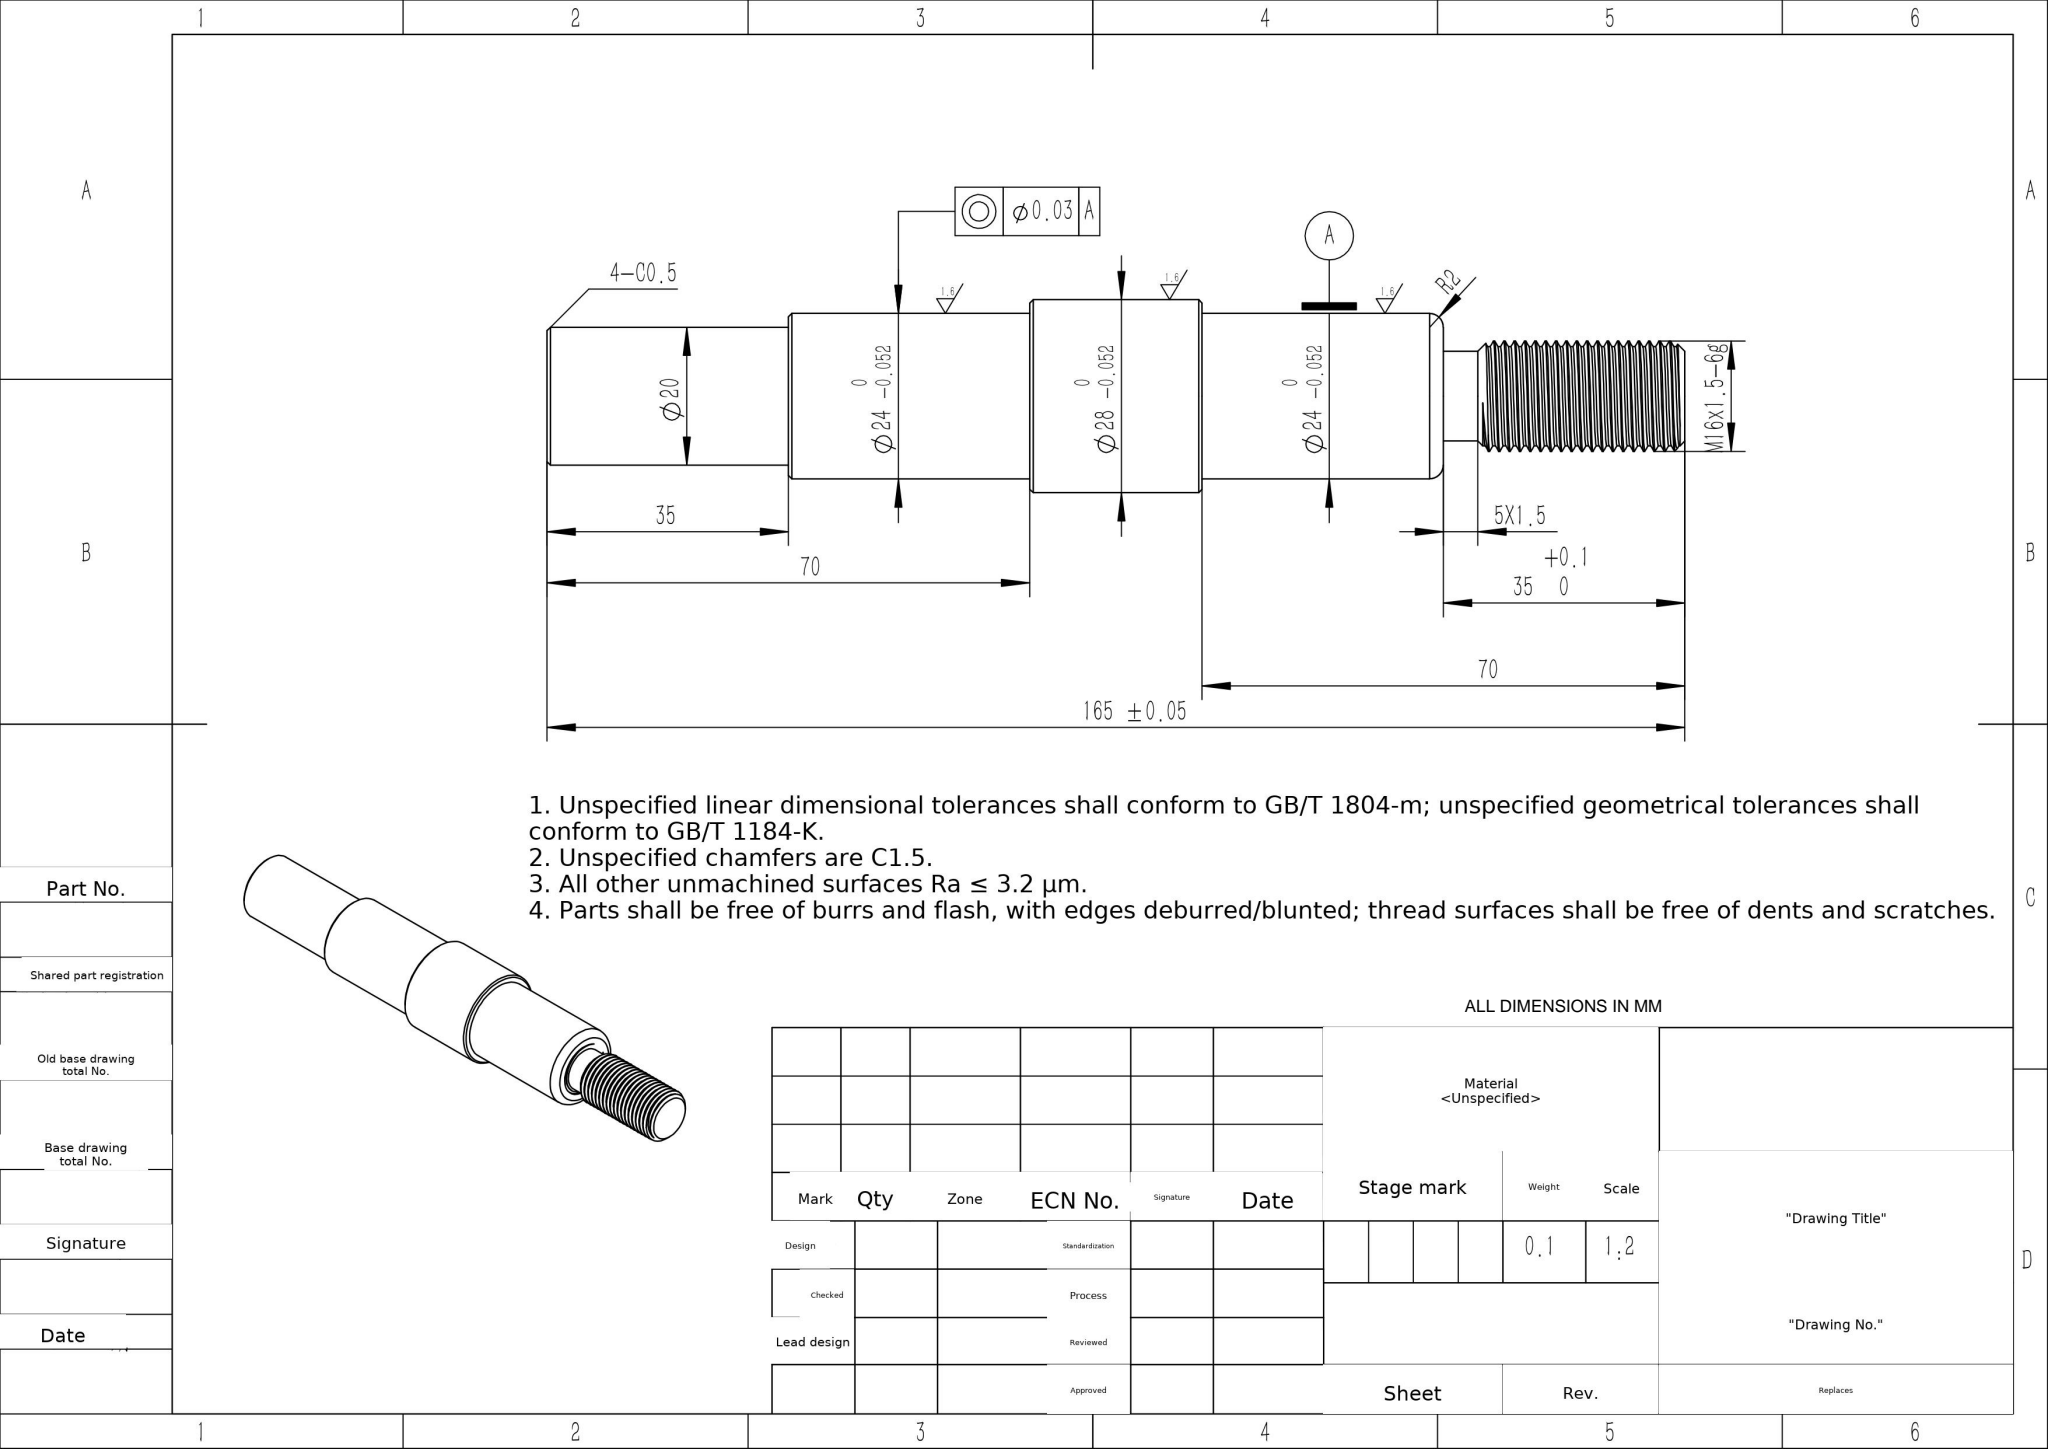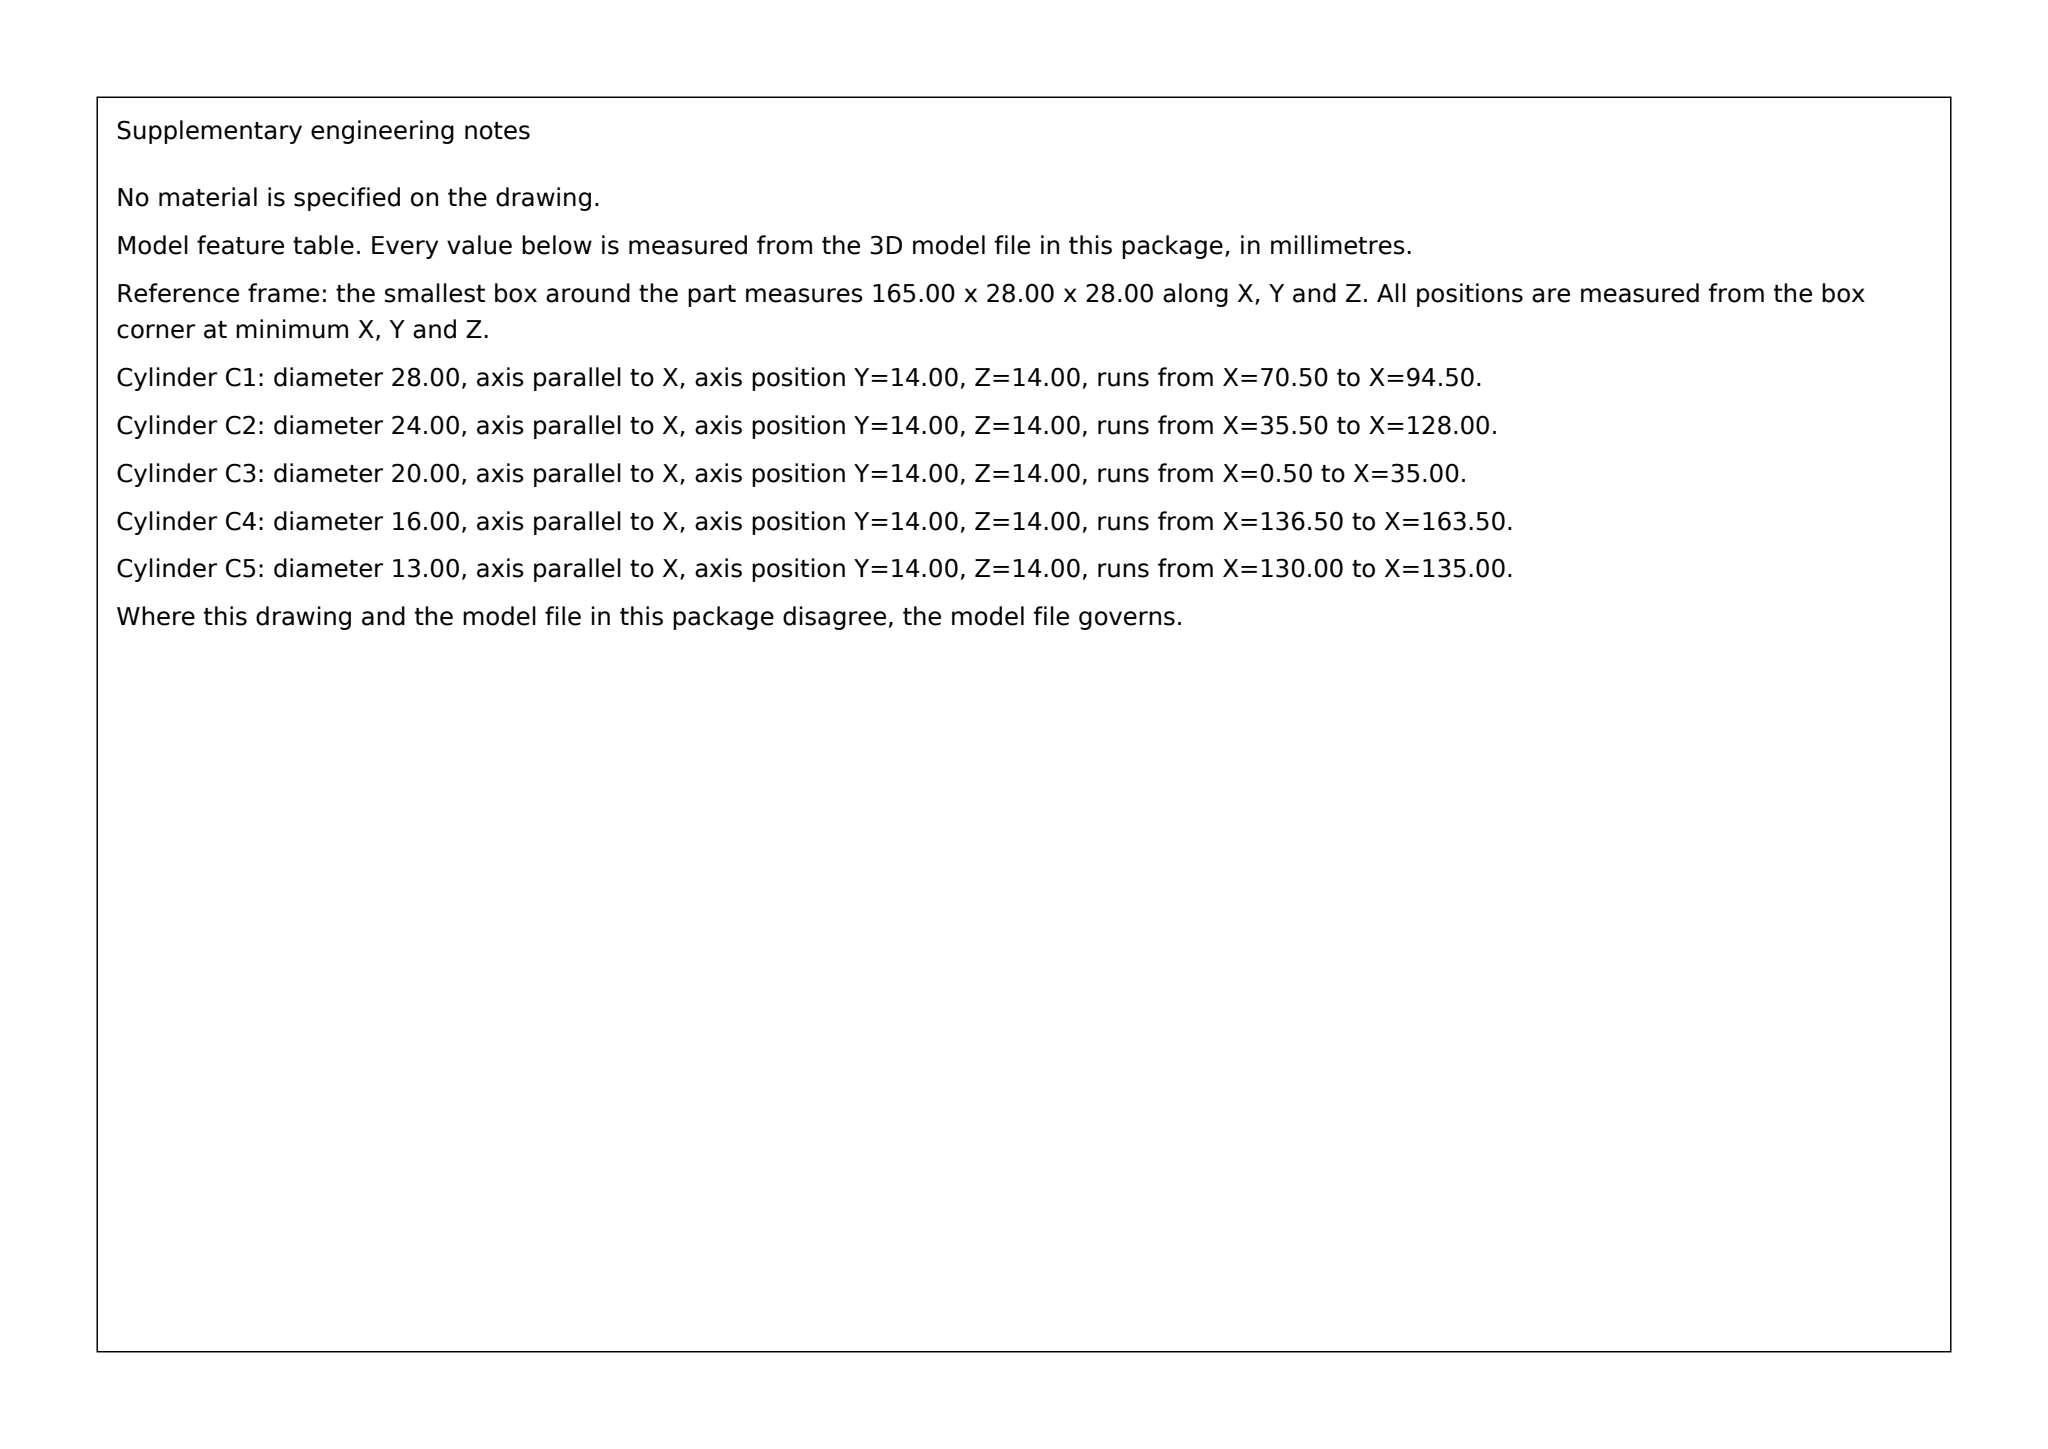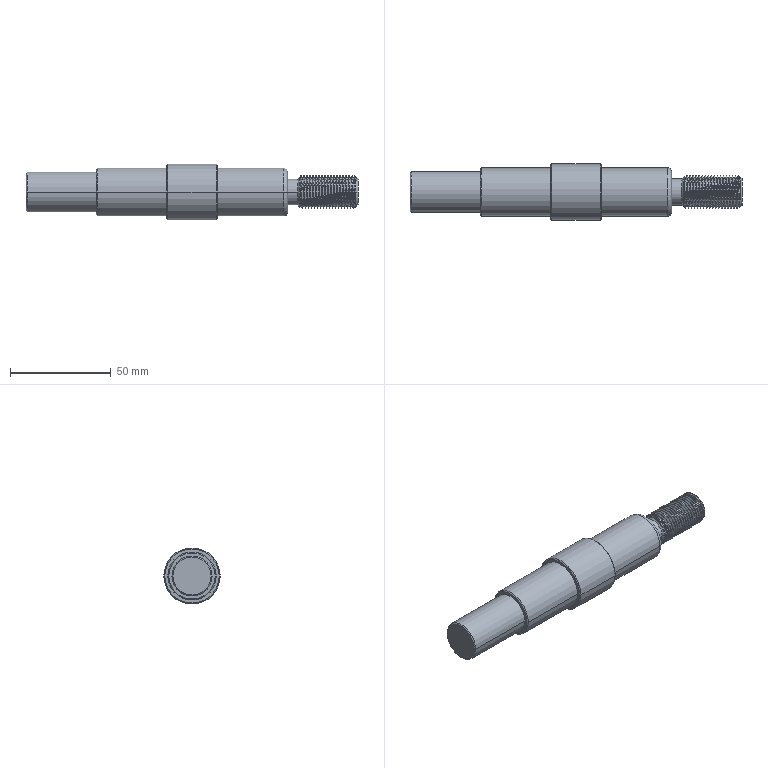Part | SolidWorks | mm | 1 solid | 75 faces | box 165 x 28 x 28 mm | volume 63826 mm3 | cylinder 47 | cone 12 | plane 7 | spline 7 | torus 2 | commonest cylinder face diameters 16 x37 24 x4 13 x2 28 x2 20 x2